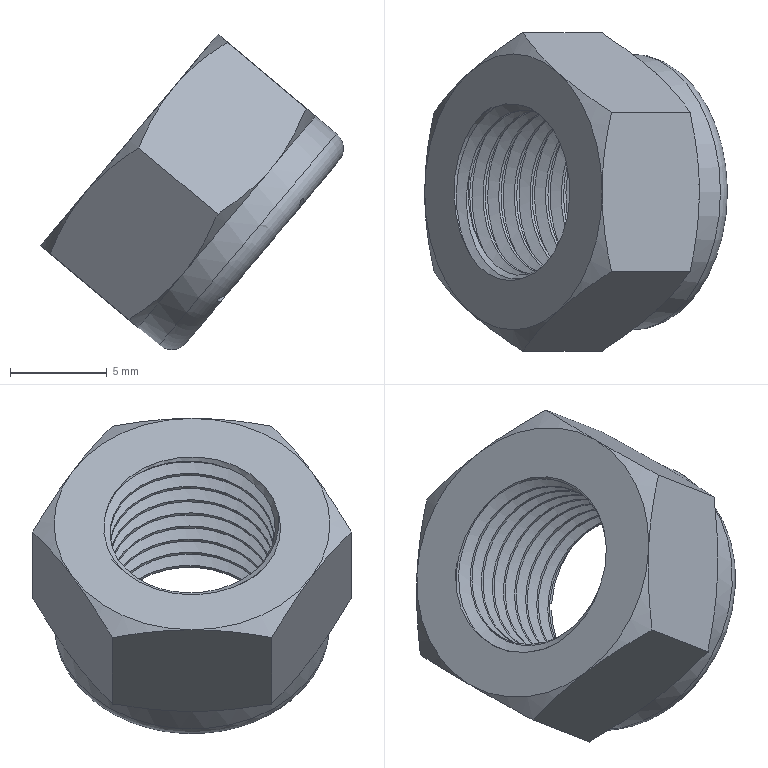Component | NX | KINGPINNUT_2 | 1 solid | 50 faces | volume 947 mm3 | plane 19 | cone 17 | cylinder 10 | spline 3 | torus 1 | commonest cylinder face diameters 0.4 x6 9.558 x2 14.287 x1 8.5 x1